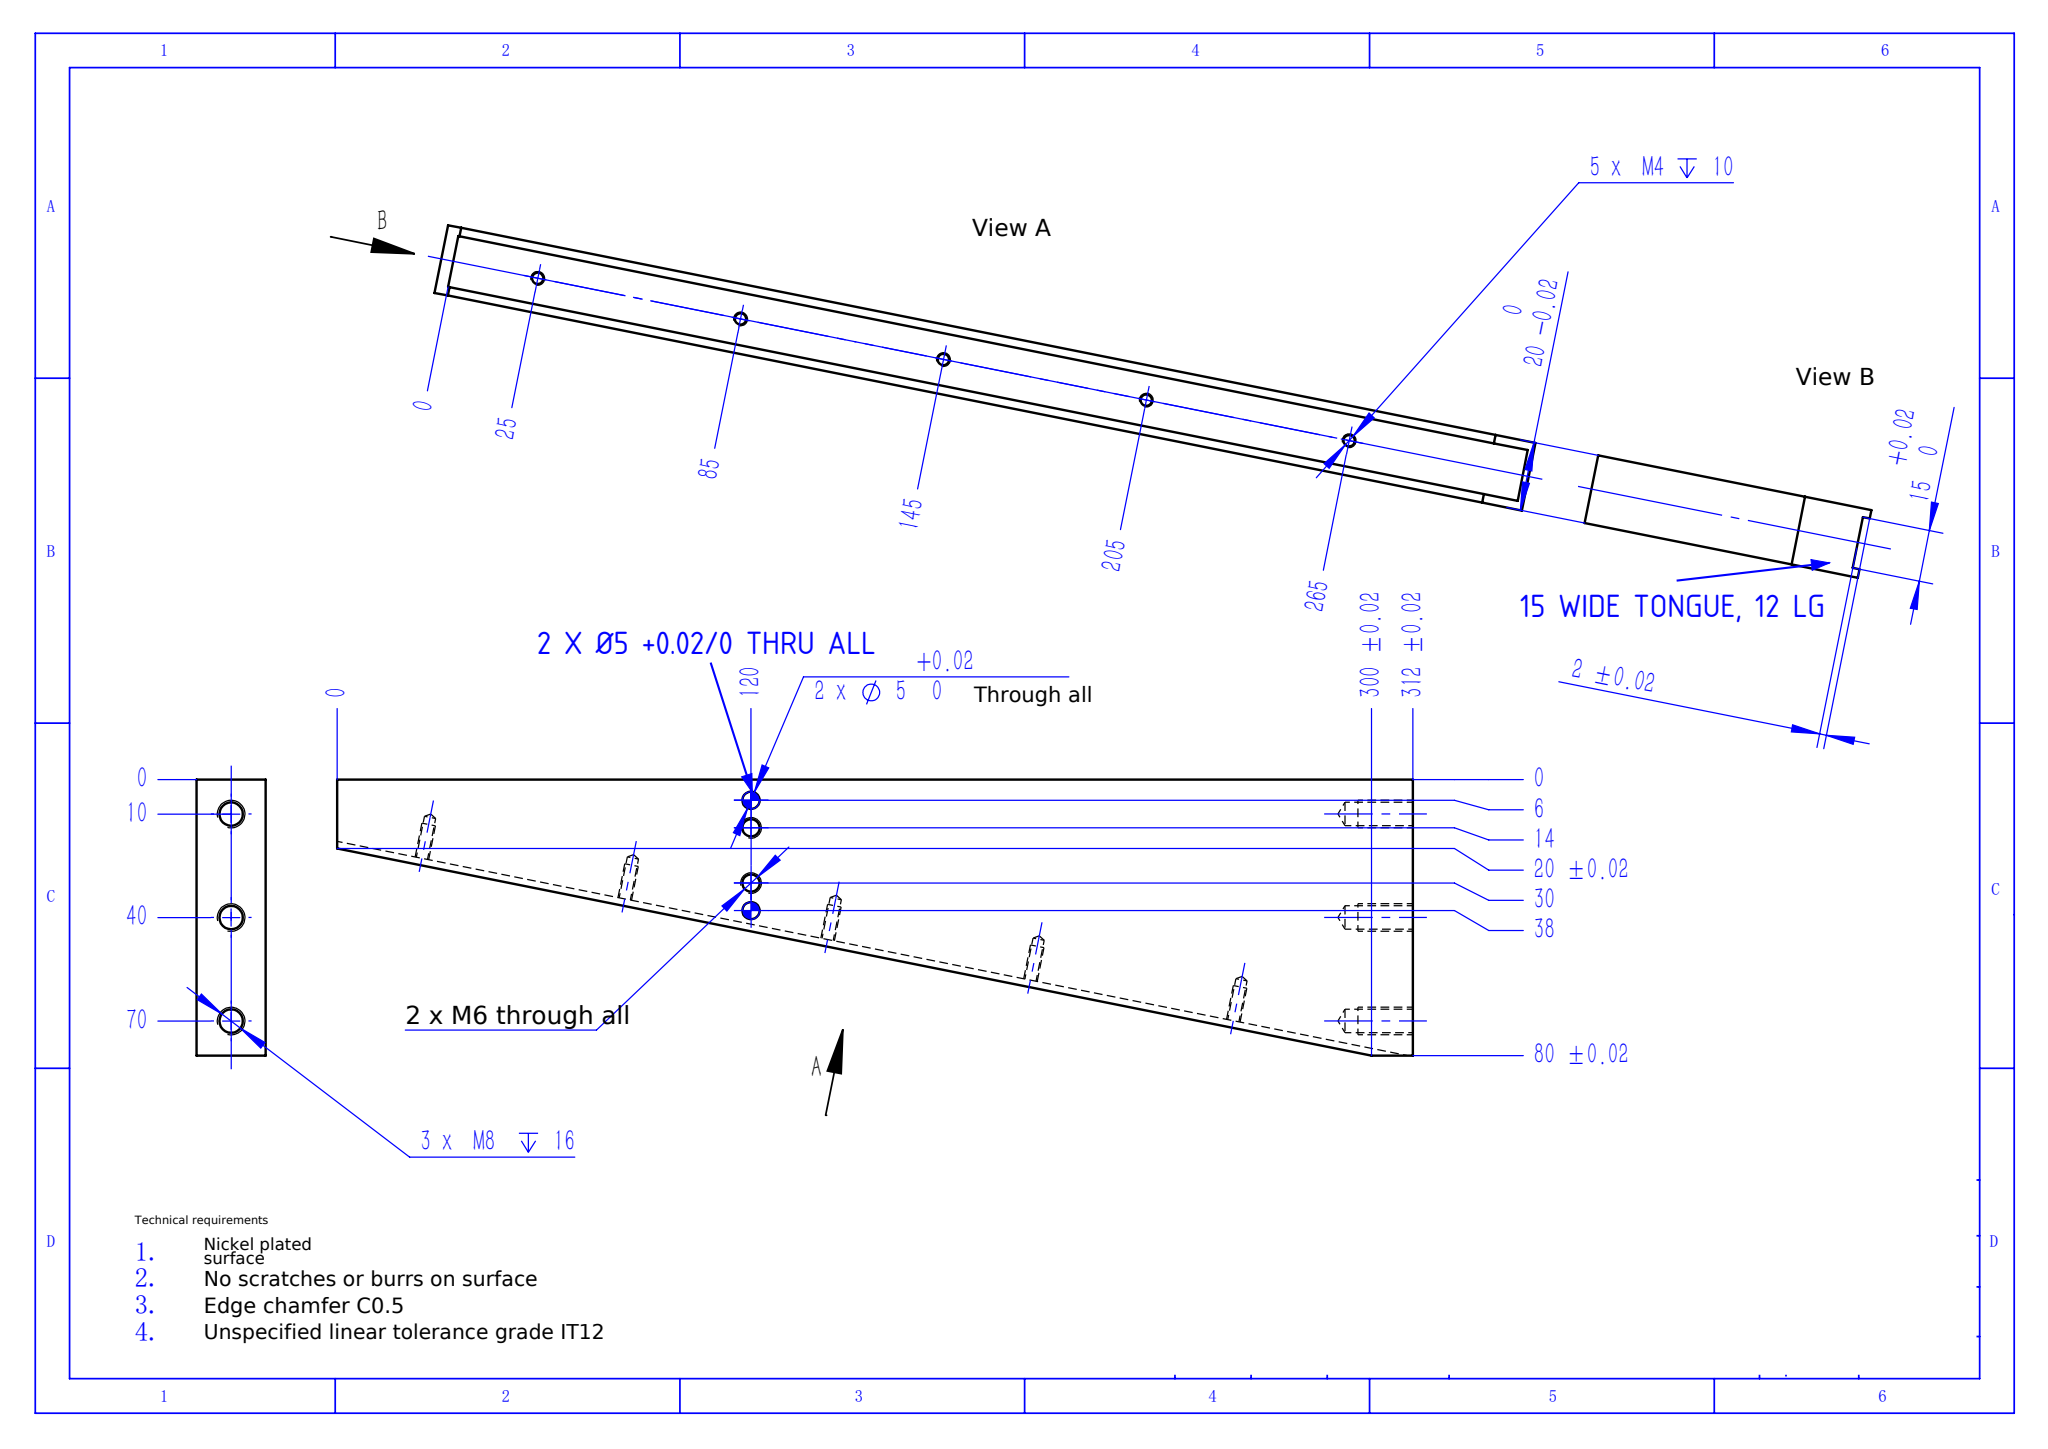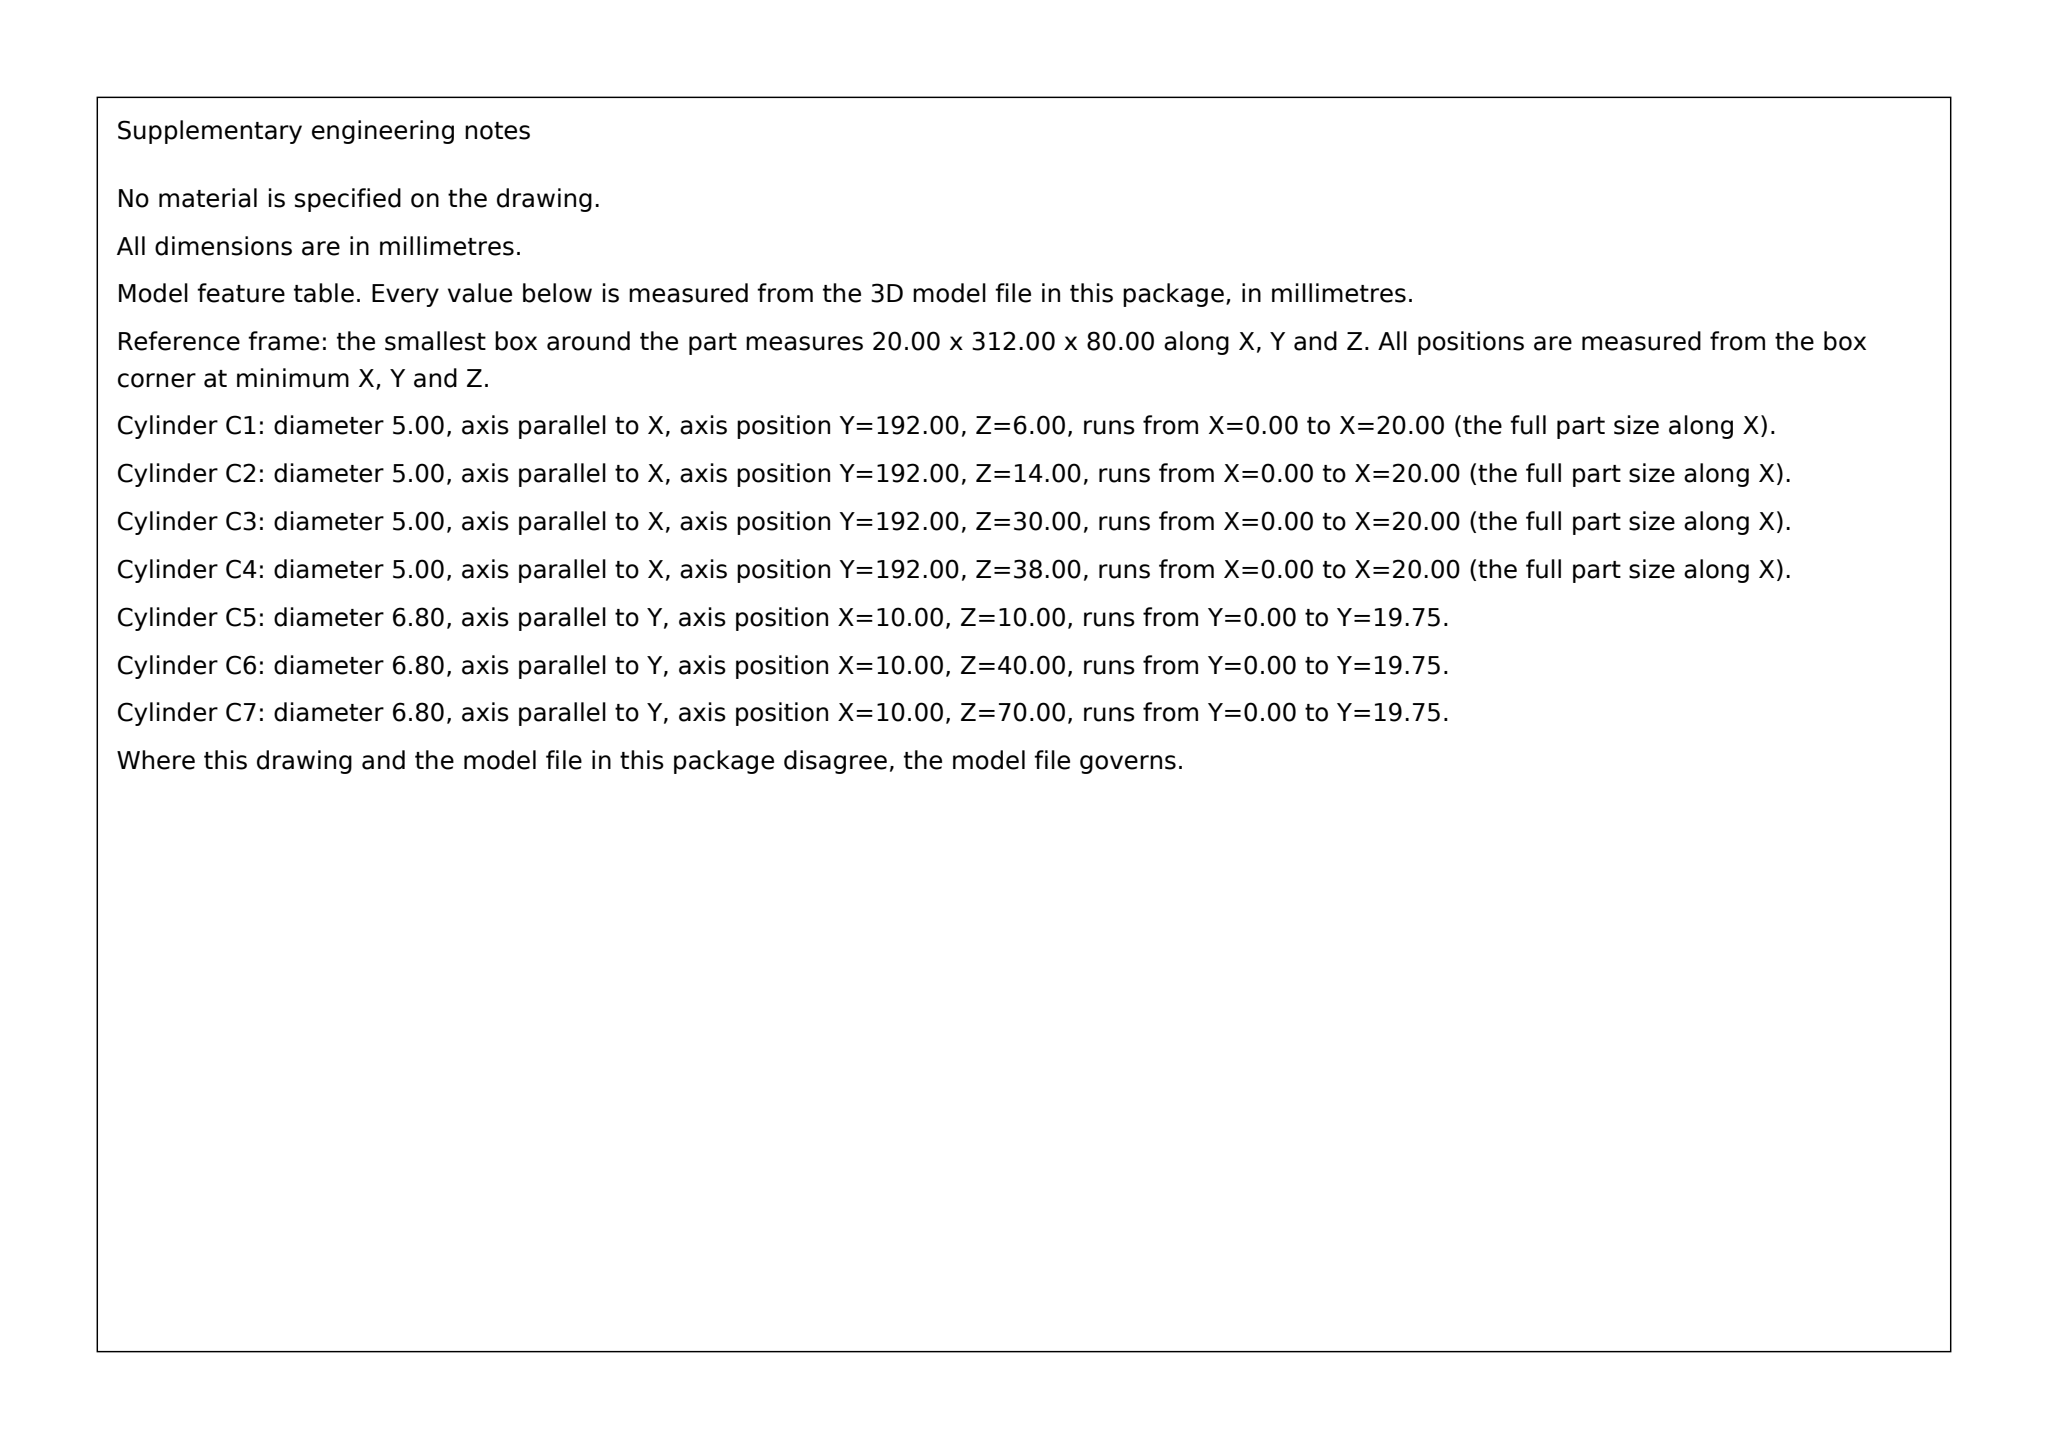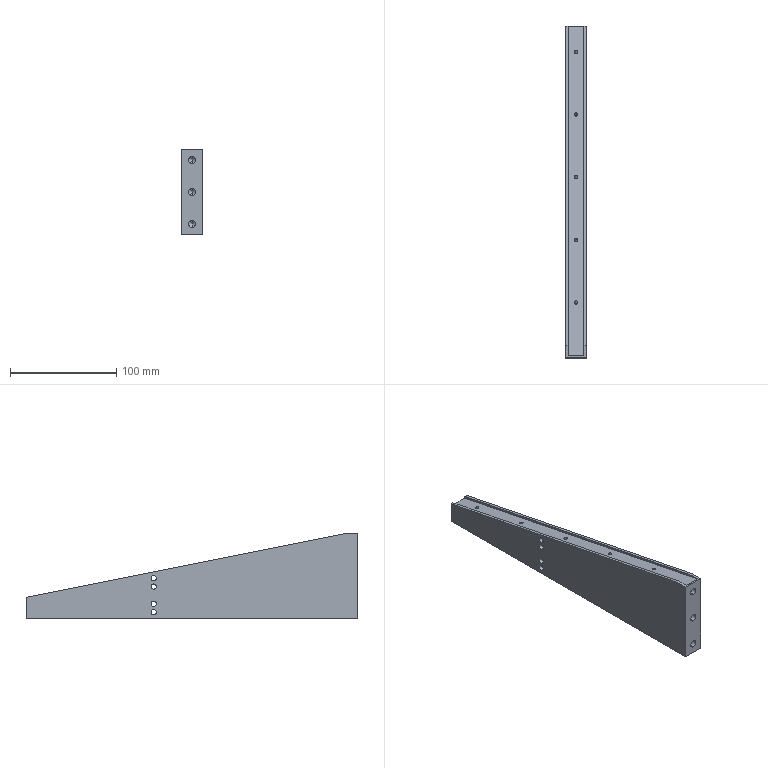Part | SolidWorks | mm | 1 solid | 51 faces | box 20 x 312 x 80 mm | volume 305537 mm3 | cylinder 24 | cone 16 | plane 11 | commonest cylinder face diameters 3.3 x10 5 x8 6.8 x6
Drawing notes:
15 WIDE TONGUE: 12 LG, Y300 TO 312 END; 2.5 STEP EA SIDE | from the solid: bbox Y=312, X=20; step faces x=2.5 & x=17.5 (17.5-2.5=15); tongue ends at Y312, body end plane at Y300 (312-300=12)
2 X Ø5 +0.02/0 THRU ALL - HOLE DIA IS Ø5 (NOT Ø50) | from the solid: cylinders dia 5.0, axis x, len 20.0 = full 20 wide part (thru all), at y=192, z=6/14/30/38